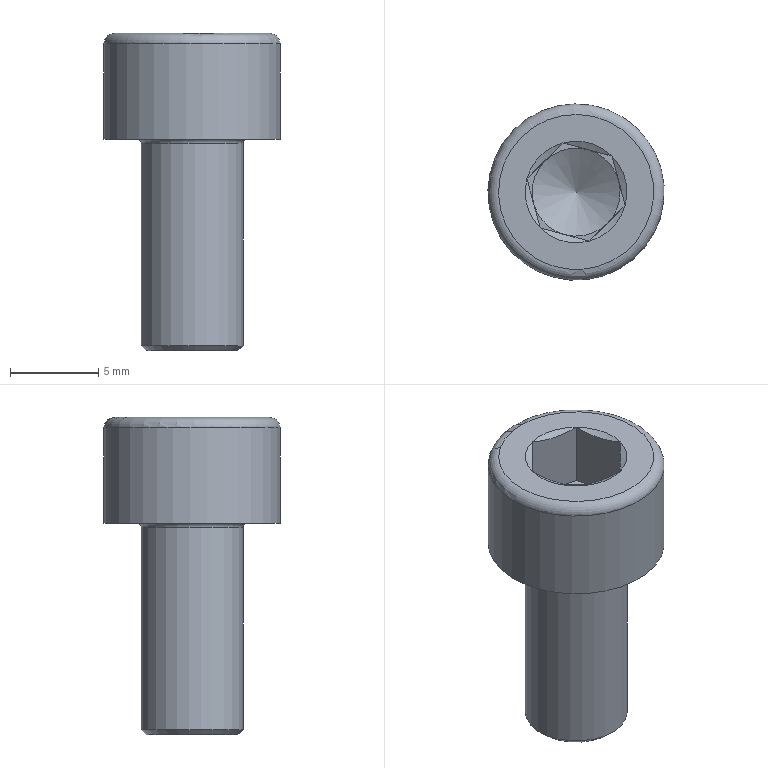Component | NX | GB-T70_1-2000_M6X12_2 | 1 solid | 27 faces | volume 695 mm3 | plane 15 | cone 8 | cylinder 2 | torus 2 | commonest cylinder face diameters 5.795 x1 10 x1